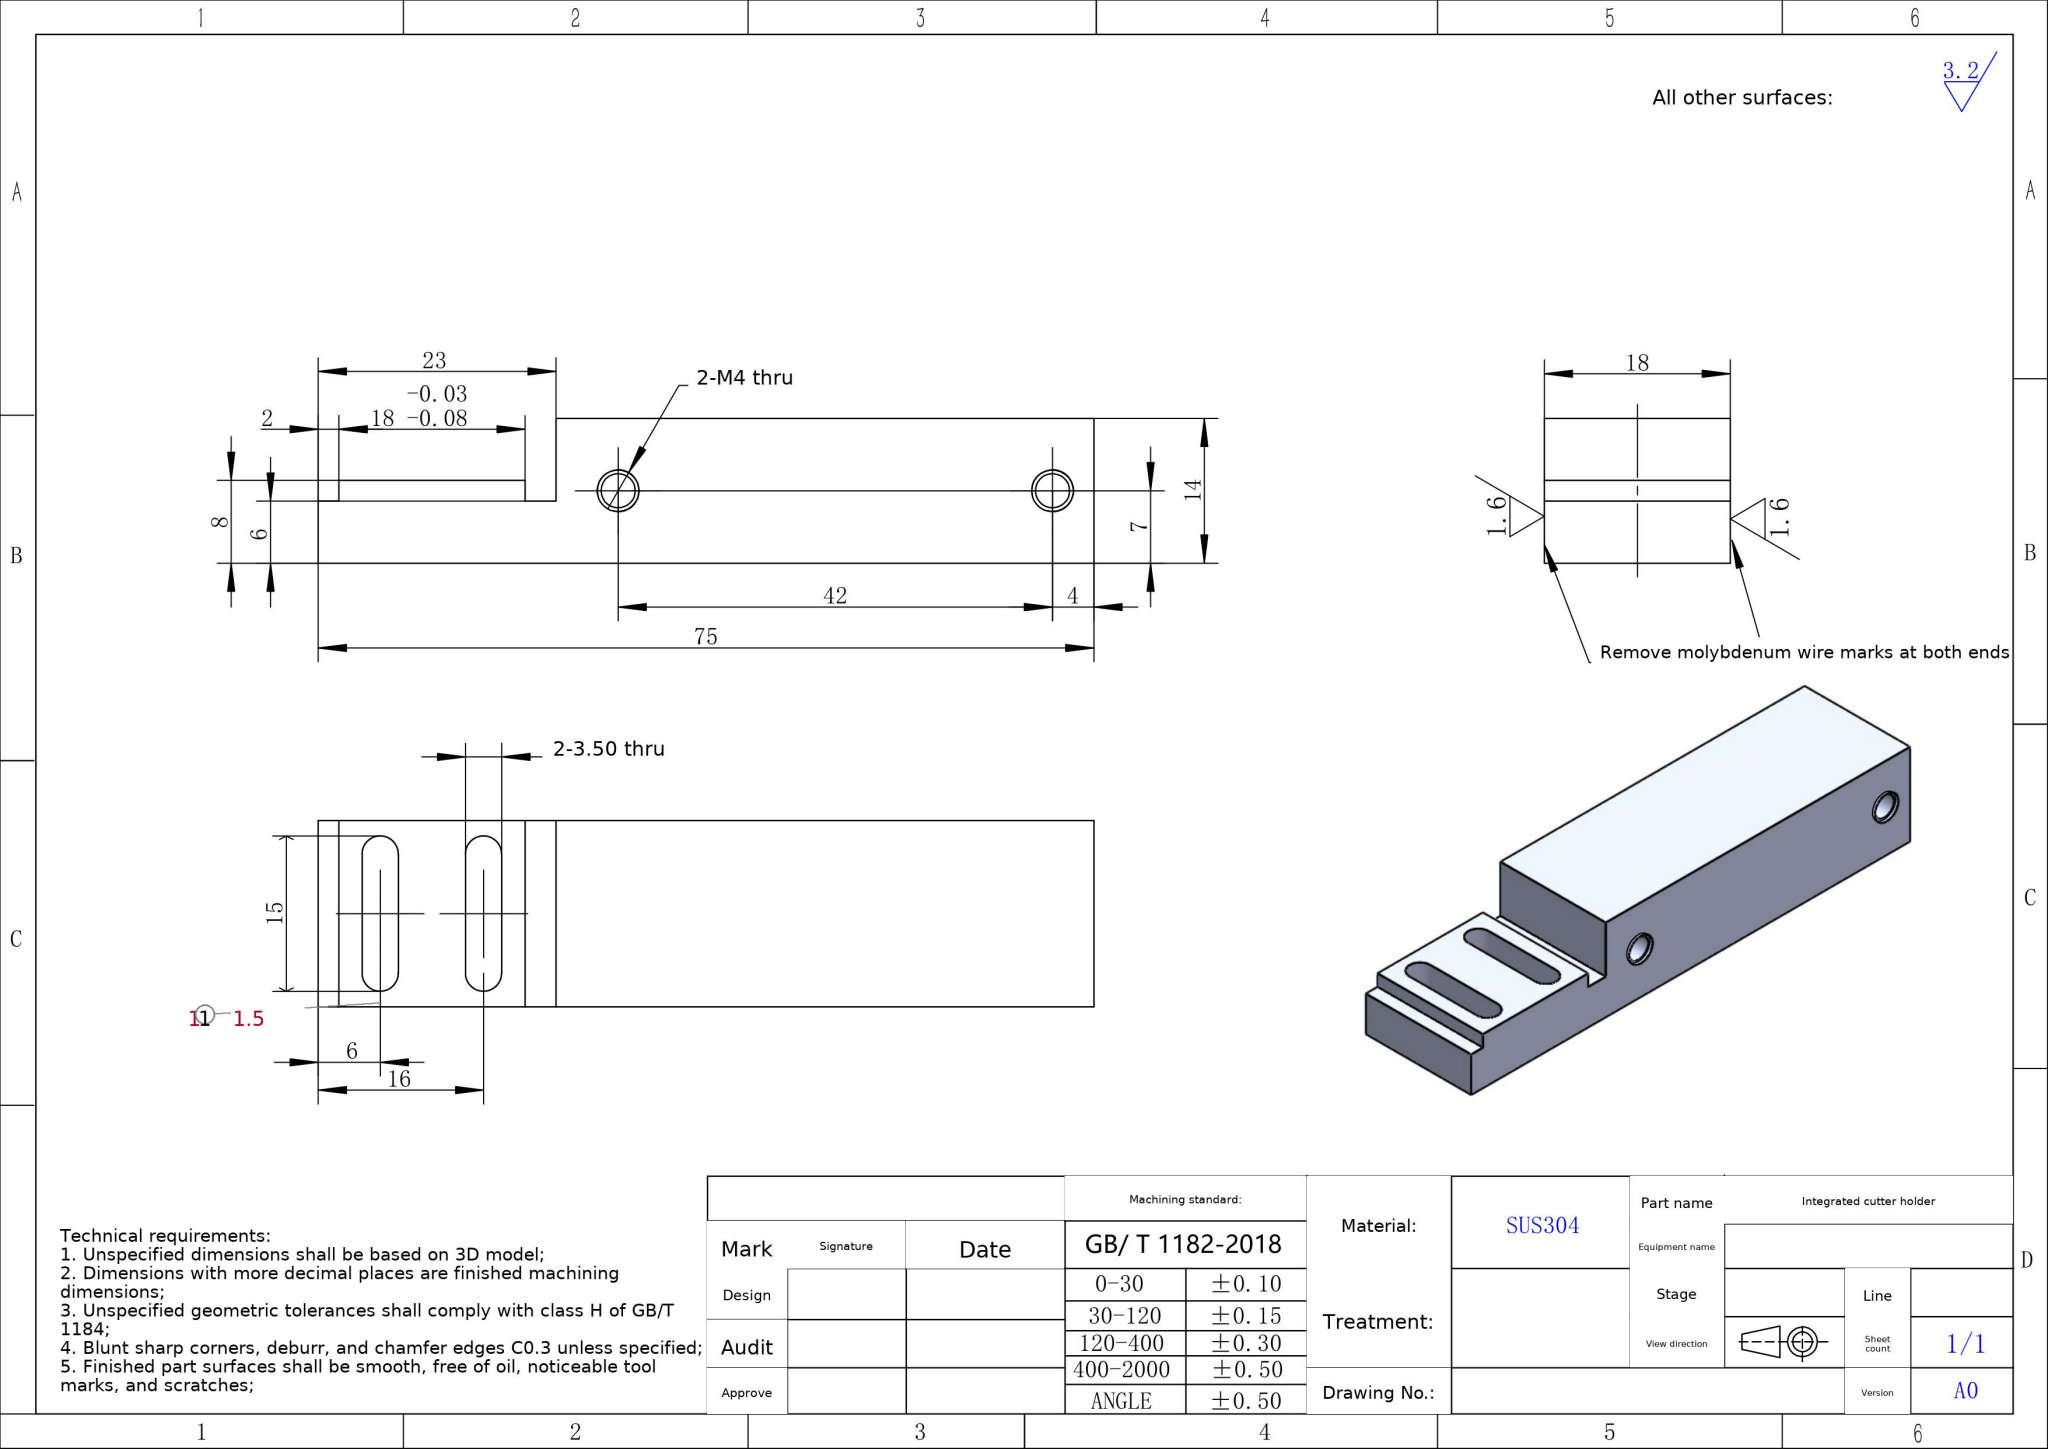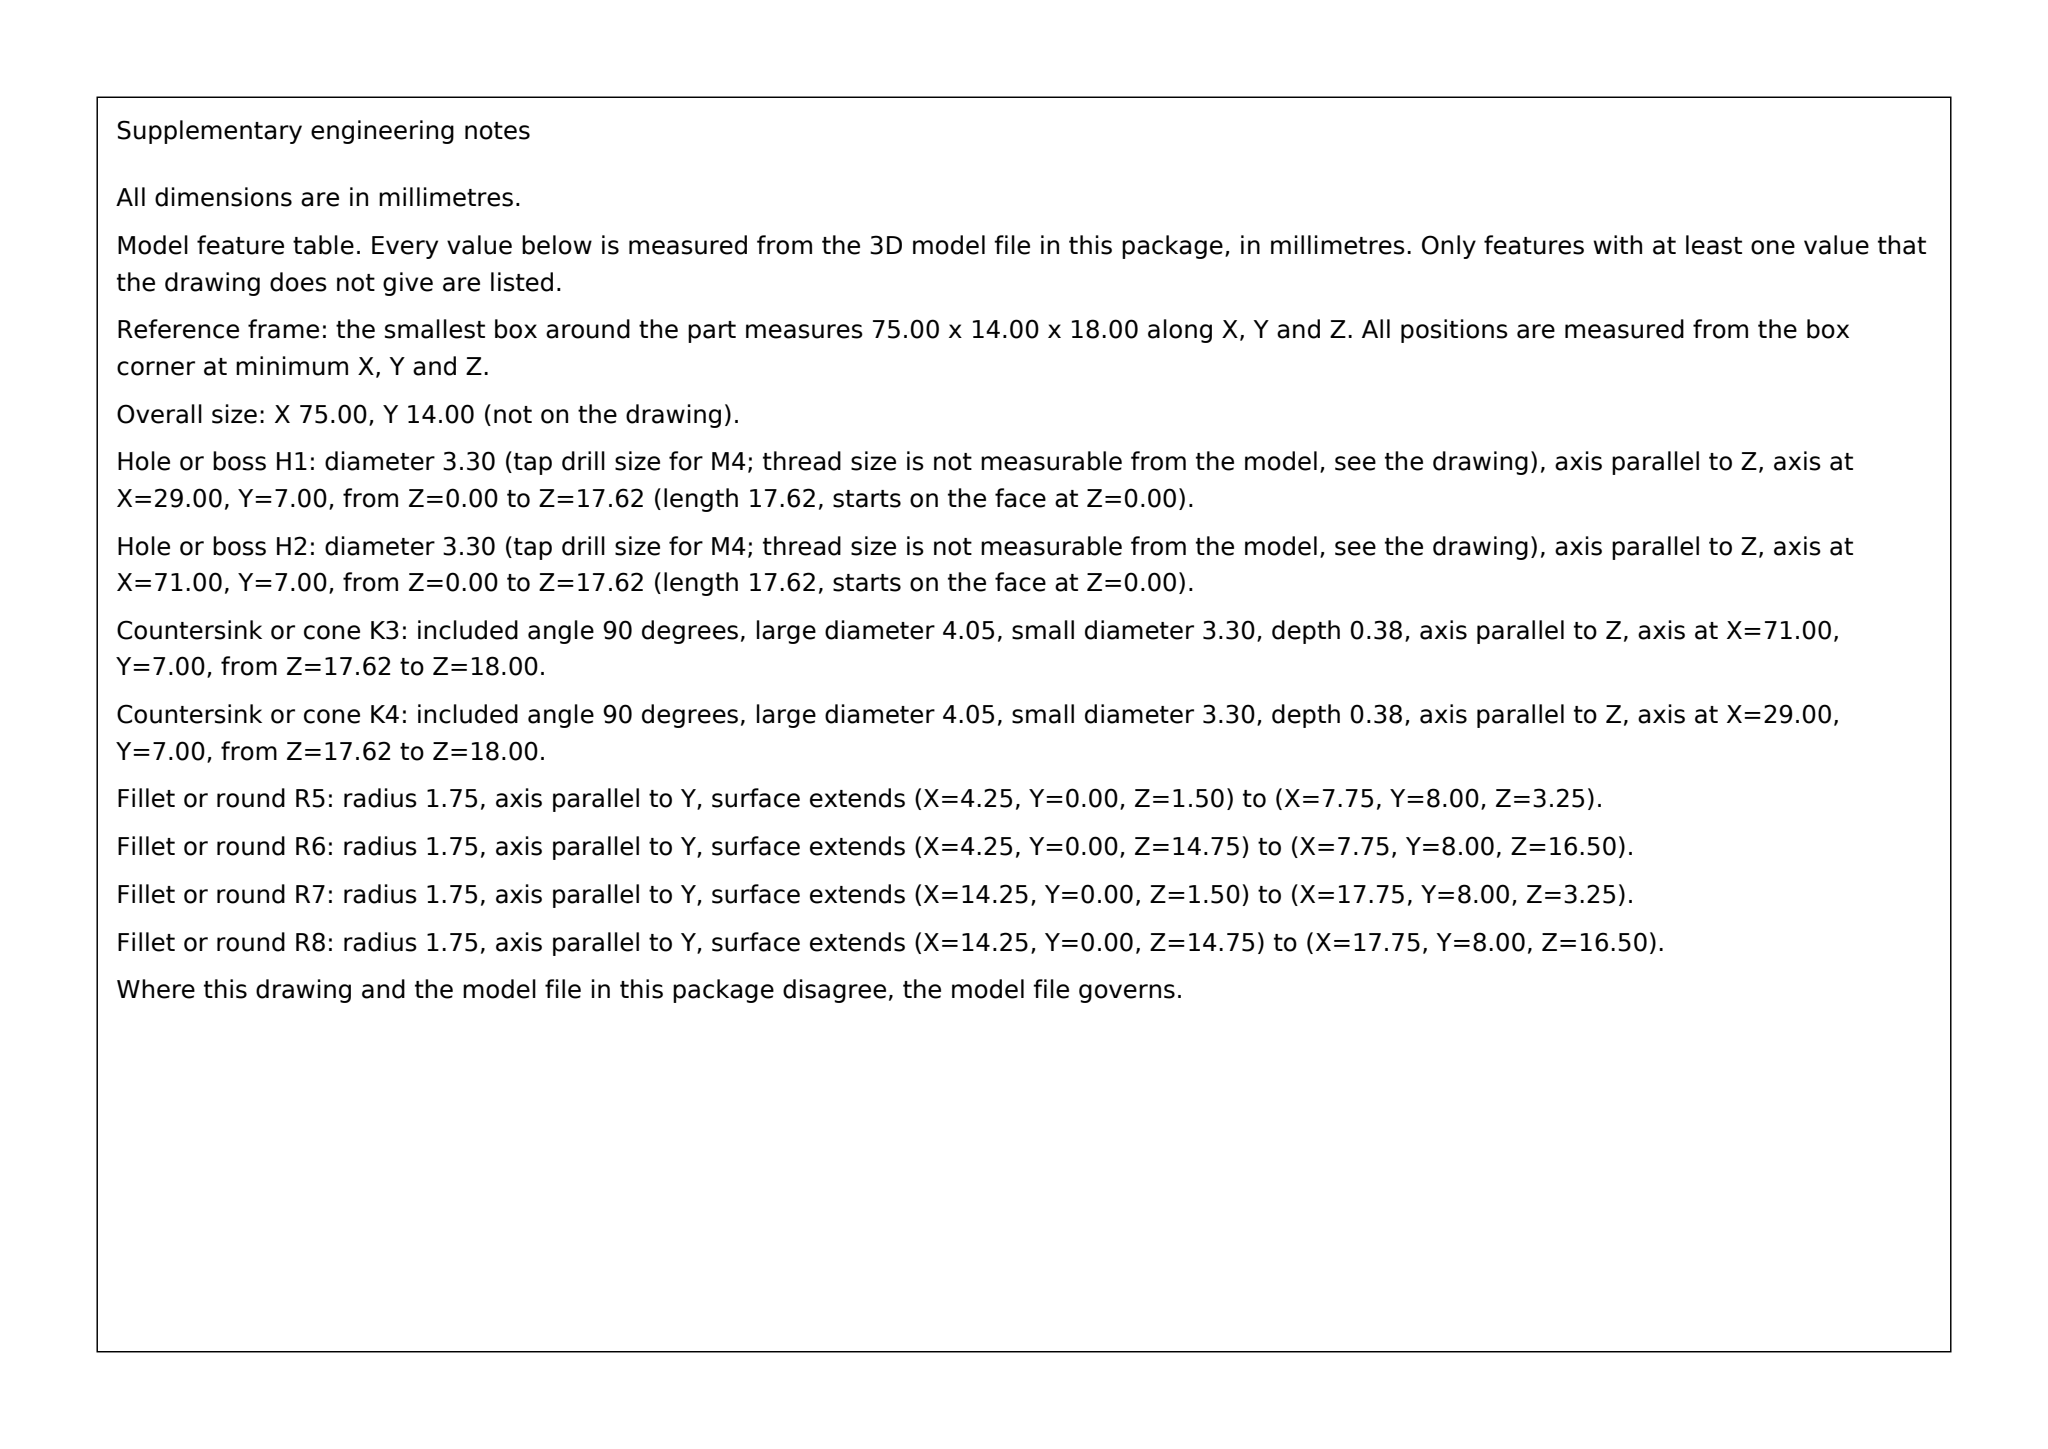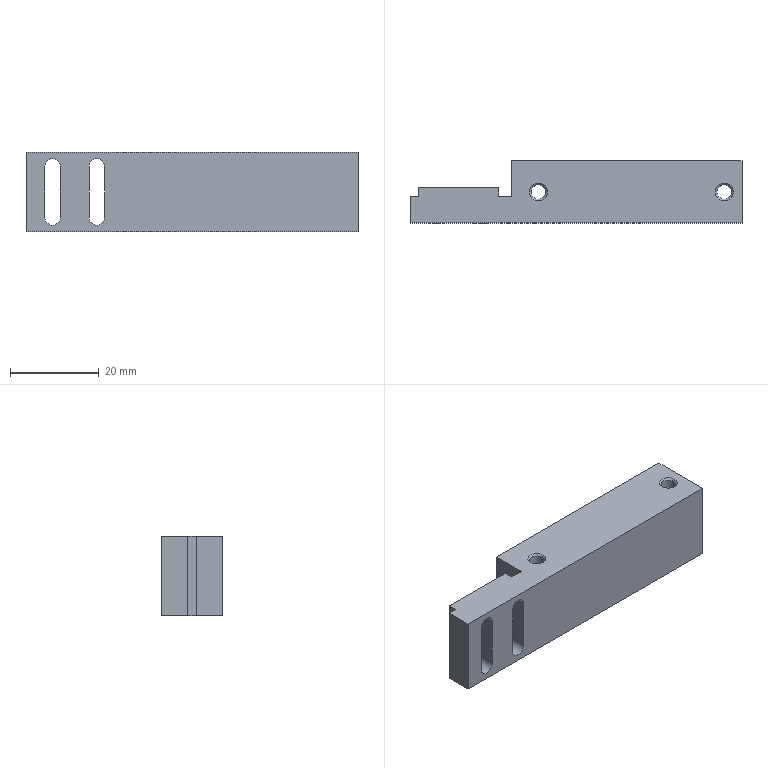Part | SolidWorks | mm | material SUS304 | 1 solid | 30 faces | box 75 x 14 x 18 mm | volume 15129 mm3 | plane 16 | cylinder 10 | cone 4 | commonest cylinder face diameters 3.5 x6 3.3 x4
build123d program:
from build123d import *

# Parameters (mm, degrees)
BOSS_EXTRUDE1_DEPTH         = 9
M4_TAPPED_HOLE1_D           = 3.3
M4_TAPPED_HOLE1_CSINK_D     = 4.05
M4_TAPPED_HOLE1_CSINK_ANGLE = 90
CUT_EXTRUDE1_DEPTH          = 76.961


with BuildPart() as part:
    # Sketch1 → Boss-Extrude1 (new, symmetric)
    with BuildSketch(Plane.XY):
        Polygon((0, 0), (0, 6), (2, 6), (2, 8), (20, 8), (20, 6), (23, 6), (23, 14), (75, 14), (75, 0), align=None)
    extrude(amount=BOSS_EXTRUDE1_DEPTH, both=True)

    # M4 Tapped Hole1 (through all)
    with Locations(Plane.XY.offset(9)):
        with Locations((71, 7), (29, 7)):
            CounterSinkHole(M4_TAPPED_HOLE1_D / 2, M4_TAPPED_HOLE1_CSINK_D / 2, counter_sink_angle=M4_TAPPED_HOLE1_CSINK_ANGLE)

    # Sketch5 → Cut-Extrude1 (cut, through all)
    with BuildSketch(Plane(origin=(0, 8, 0), x_dir=(1, 0, 0), z_dir=(0, 1, 0))):
        with BuildLine():
            Line((7.75, 5.75), (7.75, -5.75))
            ThreePointArc((7.75, -5.75), (6, -7.5), (4.25, -5.75))
            Line((4.25, -5.75), (4.25, 5.75))
            ThreePointArc((4.25, 5.75), (6, 7.5), (7.75, 5.75))
        make_face()
        with BuildLine():
            Line((17.75, 5.75), (17.75, -5.75))
            ThreePointArc((17.75, -5.75), (16, -7.5), (14.25, -5.75))
            Line((14.25, -5.75), (14.25, 5.75))
            ThreePointArc((14.25, 5.75), (16, 7.5), (17.75, 5.75))
        make_face()
    extrude(amount=-CUT_EXTRUDE1_DEPTH, mode=Mode.SUBTRACT)


solid = part.part